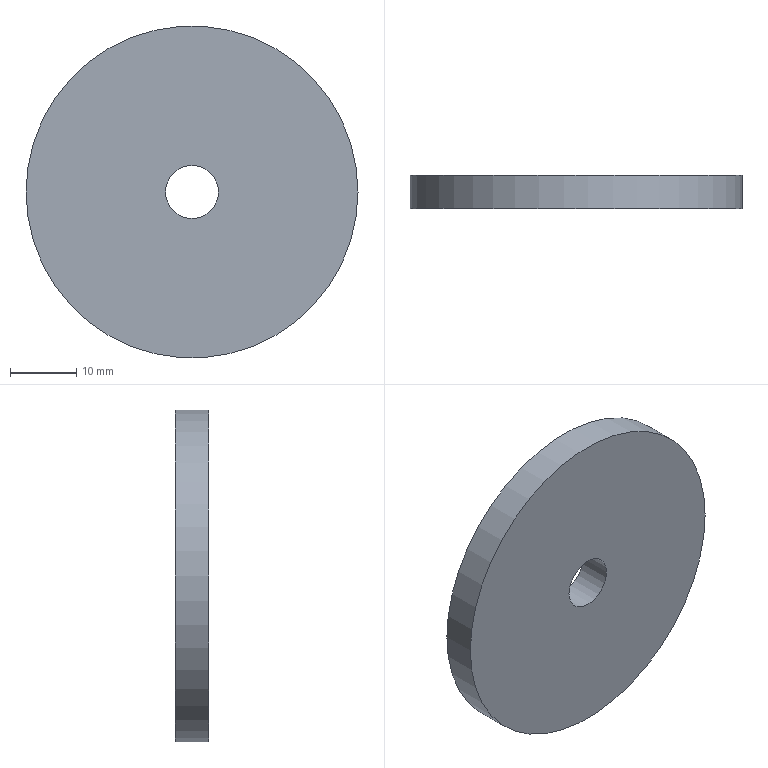Component | NX | FRONT_WHEEL | 1 solid | 4 faces | box 50 x 5 x 50 mm | volume 9566 mm3 | cylinder 2 | plane 2 | commonest cylinder face diameters 50 x1 8 x1
STEP:
#1=CARTESIAN_POINT('',(0.,0.,0.));
#2=DIRECTION('',(0.,0.,1.));
#3=DIRECTION('',(1.,0.,0.));
#4=AXIS2_PLACEMENT_3D('',#1,#2,#3);
#5=CARTESIAN_POINT('',(-218.955,2.5,-58.));
#6=VERTEX_POINT('',#5);
#7=CARTESIAN_POINT('',(-193.955,2.5,-58.));
#8=DIRECTION('',(0.,1.,0.));
#9=DIRECTION('',(-1.,0.,0.));
#10=AXIS2_PLACEMENT_3D('',#7,#8,#9);
#11=CIRCLE('',#10,25.);
#12=CARTESIAN_POINT('',(-193.955,2.5,-58.));
#13=DIRECTION('',(0.,-1.,0.));
#14=DIRECTION('',(0.,0.,1.));
#15=AXIS2_PLACEMENT_3D('',#12,#13,#14);
#16=CYLINDRICAL_SURFACE('',#15,25.);
#17=CARTESIAN_POINT('',(7.854,0.));
#18=DIRECTION('',(-1.,0.));
#19=VECTOR('',#18,1.);
#20=LINE('',#17,#19);
#21=(GEOMETRIC_REPRESENTATION_CONTEXT(2)PARAMETRIC_REPRESENTATION_CONTEXT()REPRESENTATION_CONTEXT('',''));
#22=DEFINITIONAL_REPRESENTATION('',(#20),#21);
#23=PCURVE('',#16,#22);
#24=CARTESIAN_POINT('',(-193.955,2.5,-58.));
#25=DIRECTION('',(0.,1.,0.));
#26=DIRECTION('',(0.,0.,-1.));
#27=AXIS2_PLACEMENT_3D('',#24,#25,#26);
#28=PLANE('',#27);
#29=CARTESIAN_POINT('',(0.,0.));
#30=DIRECTION('',(0.,1.));
#31=AXIS2_PLACEMENT_2D('',#29,#30);
#32=CIRCLE('',#31,25.);
#33=(GEOMETRIC_REPRESENTATION_CONTEXT(2)PARAMETRIC_REPRESENTATION_CONTEXT()REPRESENTATION_CONTEXT('',''));
#34=DEFINITIONAL_REPRESENTATION('',(#32),#33);
#35=PCURVE('',#28,#34);
#36=SURFACE_CURVE('',#11,(#23,#35),.PCURVE_S1.);
#37=EDGE_CURVE('',#6,#6,#36,.T.);
#38=ORIENTED_EDGE('',*,*,#37,.F.);
#39=CARTESIAN_POINT('',(-218.955,-2.5,-58.));
#40=VERTEX_POINT('',#39);
#41=CARTESIAN_POINT('',(-218.955,2.5,-58.));
#42=CARTESIAN_POINT('',(-218.955,-2.5,-58.));
#43=B_SPLINE_CURVE_WITH_KNOTS('',1,(#41,#42),.UNSPECIFIED.,.F.,.F.,(2,2),(0.,5.),.PIECEWISE_BEZIER_KNOTS.);
#44=CARTESIAN_POINT('',(7.854,0.));
#45=DIRECTION('',(0.,1.));
#46=VECTOR('',#45,1.);
#47=LINE('',#44,#46);
#48=(GEOMETRIC_REPRESENTATION_CONTEXT(2)PARAMETRIC_REPRESENTATION_CONTEXT()REPRESENTATION_CONTEXT('',''));
#49=DEFINITIONAL_REPRESENTATION('',(#47),#48);
#50=PCURVE('',#16,#49);
#51=CARTESIAN_POINT('',(1.571,0.));
#52=DIRECTION('',(0.,1.));
#53=VECTOR('',#52,1.);
#54=LINE('',#51,#53);
#55=(GEOMETRIC_REPRESENTATION_CONTEXT(2)PARAMETRIC_REPRESENTATION_CONTEXT()REPRESENTATION_CONTEXT('',''));
#56=DEFINITIONAL_REPRESENTATION('',(#54),#55);
#57=PCURVE('',#16,#56);
#58=SEAM_CURVE('',#43,(#50,#57),.PCURVE_S1.);
#59=EDGE_CURVE('',#6,#40,#58,.T.);
#60=ORIENTED_EDGE('',*,*,#59,.T.);
#61=CARTESIAN_POINT('',(-193.955,-2.5,-58.));
#62=DIRECTION('',(0.,1.,0.));
#63=DIRECTION('',(-1.,0.,0.));
#64=AXIS2_PLACEMENT_3D('',#61,#62,#63);
#65=CIRCLE('',#64,25.);
#66=CARTESIAN_POINT('',(7.854,5.));
#67=DIRECTION('',(-1.,0.));
#68=VECTOR('',#67,1.);
#69=LINE('',#66,#68);
#70=(GEOMETRIC_REPRESENTATION_CONTEXT(2)PARAMETRIC_REPRESENTATION_CONTEXT()REPRESENTATION_CONTEXT('',''));
#71=DEFINITIONAL_REPRESENTATION('',(#69),#70);
#72=PCURVE('',#16,#71);
#73=CARTESIAN_POINT('',(-193.955,-2.5,-58.));
#74=DIRECTION('',(0.,1.,0.));
#75=DIRECTION('',(0.,0.,-1.));
#76=AXIS2_PLACEMENT_3D('',#73,#74,#75);
#77=PLANE('',#76);
#78=CARTESIAN_POINT('',(0.,0.));
#79=DIRECTION('',(0.,1.));
#80=AXIS2_PLACEMENT_2D('',#78,#79);
#81=CIRCLE('',#80,25.);
#82=(GEOMETRIC_REPRESENTATION_CONTEXT(2)PARAMETRIC_REPRESENTATION_CONTEXT()REPRESENTATION_CONTEXT('',''));
#83=DEFINITIONAL_REPRESENTATION('',(#81),#82);
#84=PCURVE('',#77,#83);
#85=SURFACE_CURVE('',#65,(#72,#84),.PCURVE_S1.);
#86=EDGE_CURVE('',#40,#40,#85,.T.);
#87=ORIENTED_EDGE('',*,*,#86,.T.);
#88=ORIENTED_EDGE('',*,*,#59,.F.);
#89=EDGE_LOOP('',(#38,#60,#87,#88));
#90=FACE_BOUND('',#89,.T.);
#91=ADVANCED_FACE('',(#90),#16,.T.);
#92=CARTESIAN_POINT('',(-197.955,2.5,-58.));
#93=VERTEX_POINT('',#92);
#94=CARTESIAN_POINT('',(-193.955,2.5,-58.));
#95=DIRECTION('',(0.,1.,0.));
#96=DIRECTION('',(-1.,0.,0.));
#97=AXIS2_PLACEMENT_3D('',#94,#95,#96);
#98=CIRCLE('',#97,4.);
#99=CARTESIAN_POINT('',(-193.955,2.5,-58.));
#100=DIRECTION('',(0.,-1.,0.));
#101=DIRECTION('',(0.,0.,1.));
#102=AXIS2_PLACEMENT_3D('',#99,#100,#101);
#103=CYLINDRICAL_SURFACE('',#102,4.);
#104=CARTESIAN_POINT('',(7.854,0.));
#105=DIRECTION('',(-1.,0.));
#106=VECTOR('',#105,1.);
#107=LINE('',#104,#106);
#108=(GEOMETRIC_REPRESENTATION_CONTEXT(2)PARAMETRIC_REPRESENTATION_CONTEXT()REPRESENTATION_CONTEXT('',''));
#109=DEFINITIONAL_REPRESENTATION('',(#107),#108);
#110=PCURVE('',#103,#109);
#111=CARTESIAN_POINT('',(0.,0.));
#112=DIRECTION('',(0.,1.));
#113=AXIS2_PLACEMENT_2D('',#111,#112);
#114=CIRCLE('',#113,4.);
#115=(GEOMETRIC_REPRESENTATION_CONTEXT(2)PARAMETRIC_REPRESENTATION_CONTEXT()REPRESENTATION_CONTEXT('',''));
#116=DEFINITIONAL_REPRESENTATION('',(#114),#115);
#117=PCURVE('',#28,#116);
#118=SURFACE_CURVE('',#98,(#110,#117),.PCURVE_S1.);
#119=EDGE_CURVE('',#93,#93,#118,.T.);
#120=ORIENTED_EDGE('',*,*,#119,.F.);
#121=CARTESIAN_POINT('',(-197.955,-2.5,-58.));
#122=VERTEX_POINT('',#121);
#123=CARTESIAN_POINT('',(-197.955,2.5,-58.));
#124=CARTESIAN_POINT('',(-197.955,-2.5,-58.));
#125=B_SPLINE_CURVE_WITH_KNOTS('',1,(#123,#124),.UNSPECIFIED.,.F.,.F.,(2,2),(0.,5.),.PIECEWISE_BEZIER_KNOTS.);
#126=CARTESIAN_POINT('',(7.854,0.));
#127=DIRECTION('',(0.,1.));
#128=VECTOR('',#127,1.);
#129=LINE('',#126,#128);
#130=(GEOMETRIC_REPRESENTATION_CONTEXT(2)PARAMETRIC_REPRESENTATION_CONTEXT()REPRESENTATION_CONTEXT('',''));
#131=DEFINITIONAL_REPRESENTATION('',(#129),#130);
#132=PCURVE('',#103,#131);
#133=CARTESIAN_POINT('',(1.571,0.));
#134=DIRECTION('',(0.,1.));
#135=VECTOR('',#134,1.);
#136=LINE('',#133,#135);
#137=(GEOMETRIC_REPRESENTATION_CONTEXT(2)PARAMETRIC_REPRESENTATION_CONTEXT()REPRESENTATION_CONTEXT('',''));
#138=DEFINITIONAL_REPRESENTATION('',(#136),#137);
#139=PCURVE('',#103,#138);
#140=SEAM_CURVE('',#125,(#132,#139),.PCURVE_S1.);
#141=EDGE_CURVE('',#93,#122,#140,.T.);
#142=ORIENTED_EDGE('',*,*,#141,.T.);
#143=CARTESIAN_POINT('',(-193.955,-2.5,-58.));
#144=DIRECTION('',(0.,1.,0.));
#145=DIRECTION('',(-1.,0.,0.));
#146=AXIS2_PLACEMENT_3D('',#143,#144,#145);
#147=CIRCLE('',#146,4.);
#148=CARTESIAN_POINT('',(7.854,5.));
#149=DIRECTION('',(-1.,0.));
#150=VECTOR('',#149,1.);
#151=LINE('',#148,#150);
#152=(GEOMETRIC_REPRESENTATION_CONTEXT(2)PARAMETRIC_REPRESENTATION_CONTEXT()REPRESENTATION_CONTEXT('',''));
#153=DEFINITIONAL_REPRESENTATION('',(#151),#152);
#154=PCURVE('',#103,#153);
#155=CARTESIAN_POINT('',(0.,0.));
#156=DIRECTION('',(0.,1.));
#157=AXIS2_PLACEMENT_2D('',#155,#156);
#158=CIRCLE('',#157,4.);
#159=(GEOMETRIC_REPRESENTATION_CONTEXT(2)PARAMETRIC_REPRESENTATION_CONTEXT()REPRESENTATION_CONTEXT('',''));
#160=DEFINITIONAL_REPRESENTATION('',(#158),#159);
#161=PCURVE('',#77,#160);
#162=SURFACE_CURVE('',#147,(#154,#161),.PCURVE_S1.);
#163=EDGE_CURVE('',#122,#122,#162,.T.);
#164=ORIENTED_EDGE('',*,*,#163,.T.);
#165=ORIENTED_EDGE('',*,*,#141,.F.);
#166=EDGE_LOOP('',(#120,#142,#164,#165));
#167=FACE_BOUND('',#166,.F.);
#168=ADVANCED_FACE('',(#167),#103,.F.);
#169=ORIENTED_EDGE('',*,*,#37,.T.);
#170=EDGE_LOOP('',(#169));
#171=FACE_BOUND('',#170,.T.);
#172=ORIENTED_EDGE('',*,*,#119,.F.);
#173=EDGE_LOOP('',(#172));
#174=FACE_BOUND('',#173,.T.);
#175=ADVANCED_FACE('',(#171,#174),#28,.T.);
#176=ORIENTED_EDGE('',*,*,#86,.F.);
#177=EDGE_LOOP('',(#176));
#178=FACE_BOUND('',#177,.T.);
#179=ORIENTED_EDGE('',*,*,#163,.T.);
#180=EDGE_LOOP('',(#179));
#181=FACE_BOUND('',#180,.T.);
#182=ADVANCED_FACE('',(#178,#181),#77,.F.);
#183=CLOSED_SHELL('',(#91,#168,#175,#182));
#184=MANIFOLD_SOLID_BREP('',#183);
#185=(LENGTH_UNIT()NAMED_UNIT(*)SI_UNIT(.MILLI.,.METRE.));
#186=UNCERTAINTY_MEASURE_WITH_UNIT(LENGTH_MEASURE(0.00001),#185,'','');
#187=(NAMED_UNIT(*)PLANE_ANGLE_UNIT()SI_UNIT($,.RADIAN.));
#188=(NAMED_UNIT(*)SI_UNIT($,.STERADIAN.)SOLID_ANGLE_UNIT());
#189=(GEOMETRIC_REPRESENTATION_CONTEXT(3)GLOBAL_UNCERTAINTY_ASSIGNED_CONTEXT((#186))GLOBAL_UNIT_ASSIGNED_CONTEXT((#185,#187,#188))REPRESENTATION_CONTEXT('',''));
#190=ADVANCED_BREP_SHAPE_REPRESENTATION('',(#4,#184),#189);